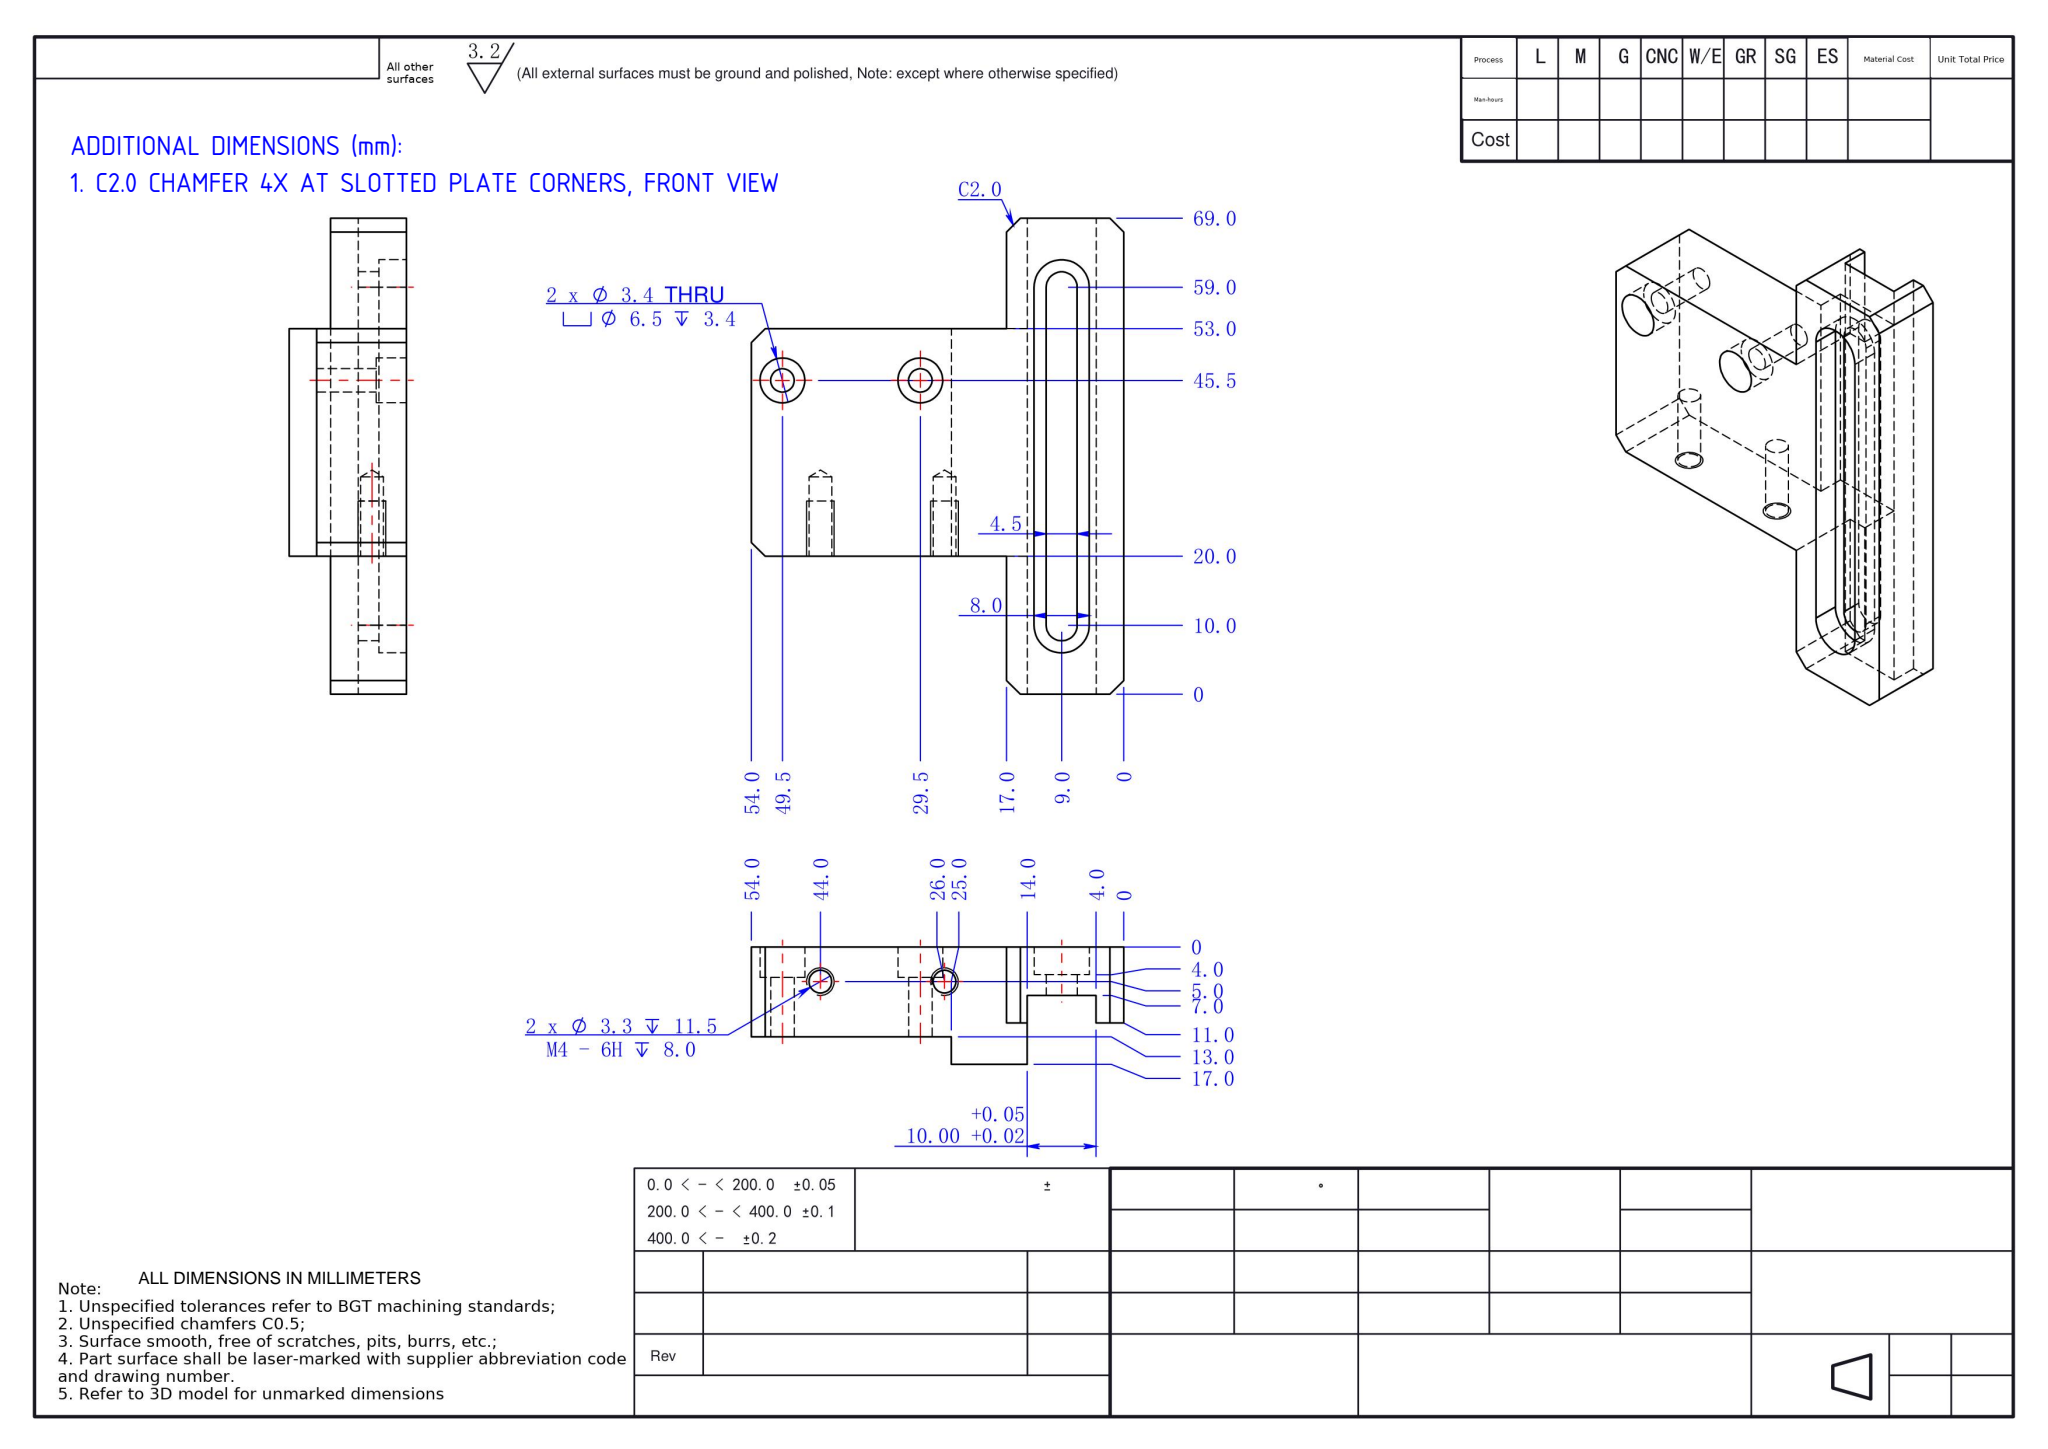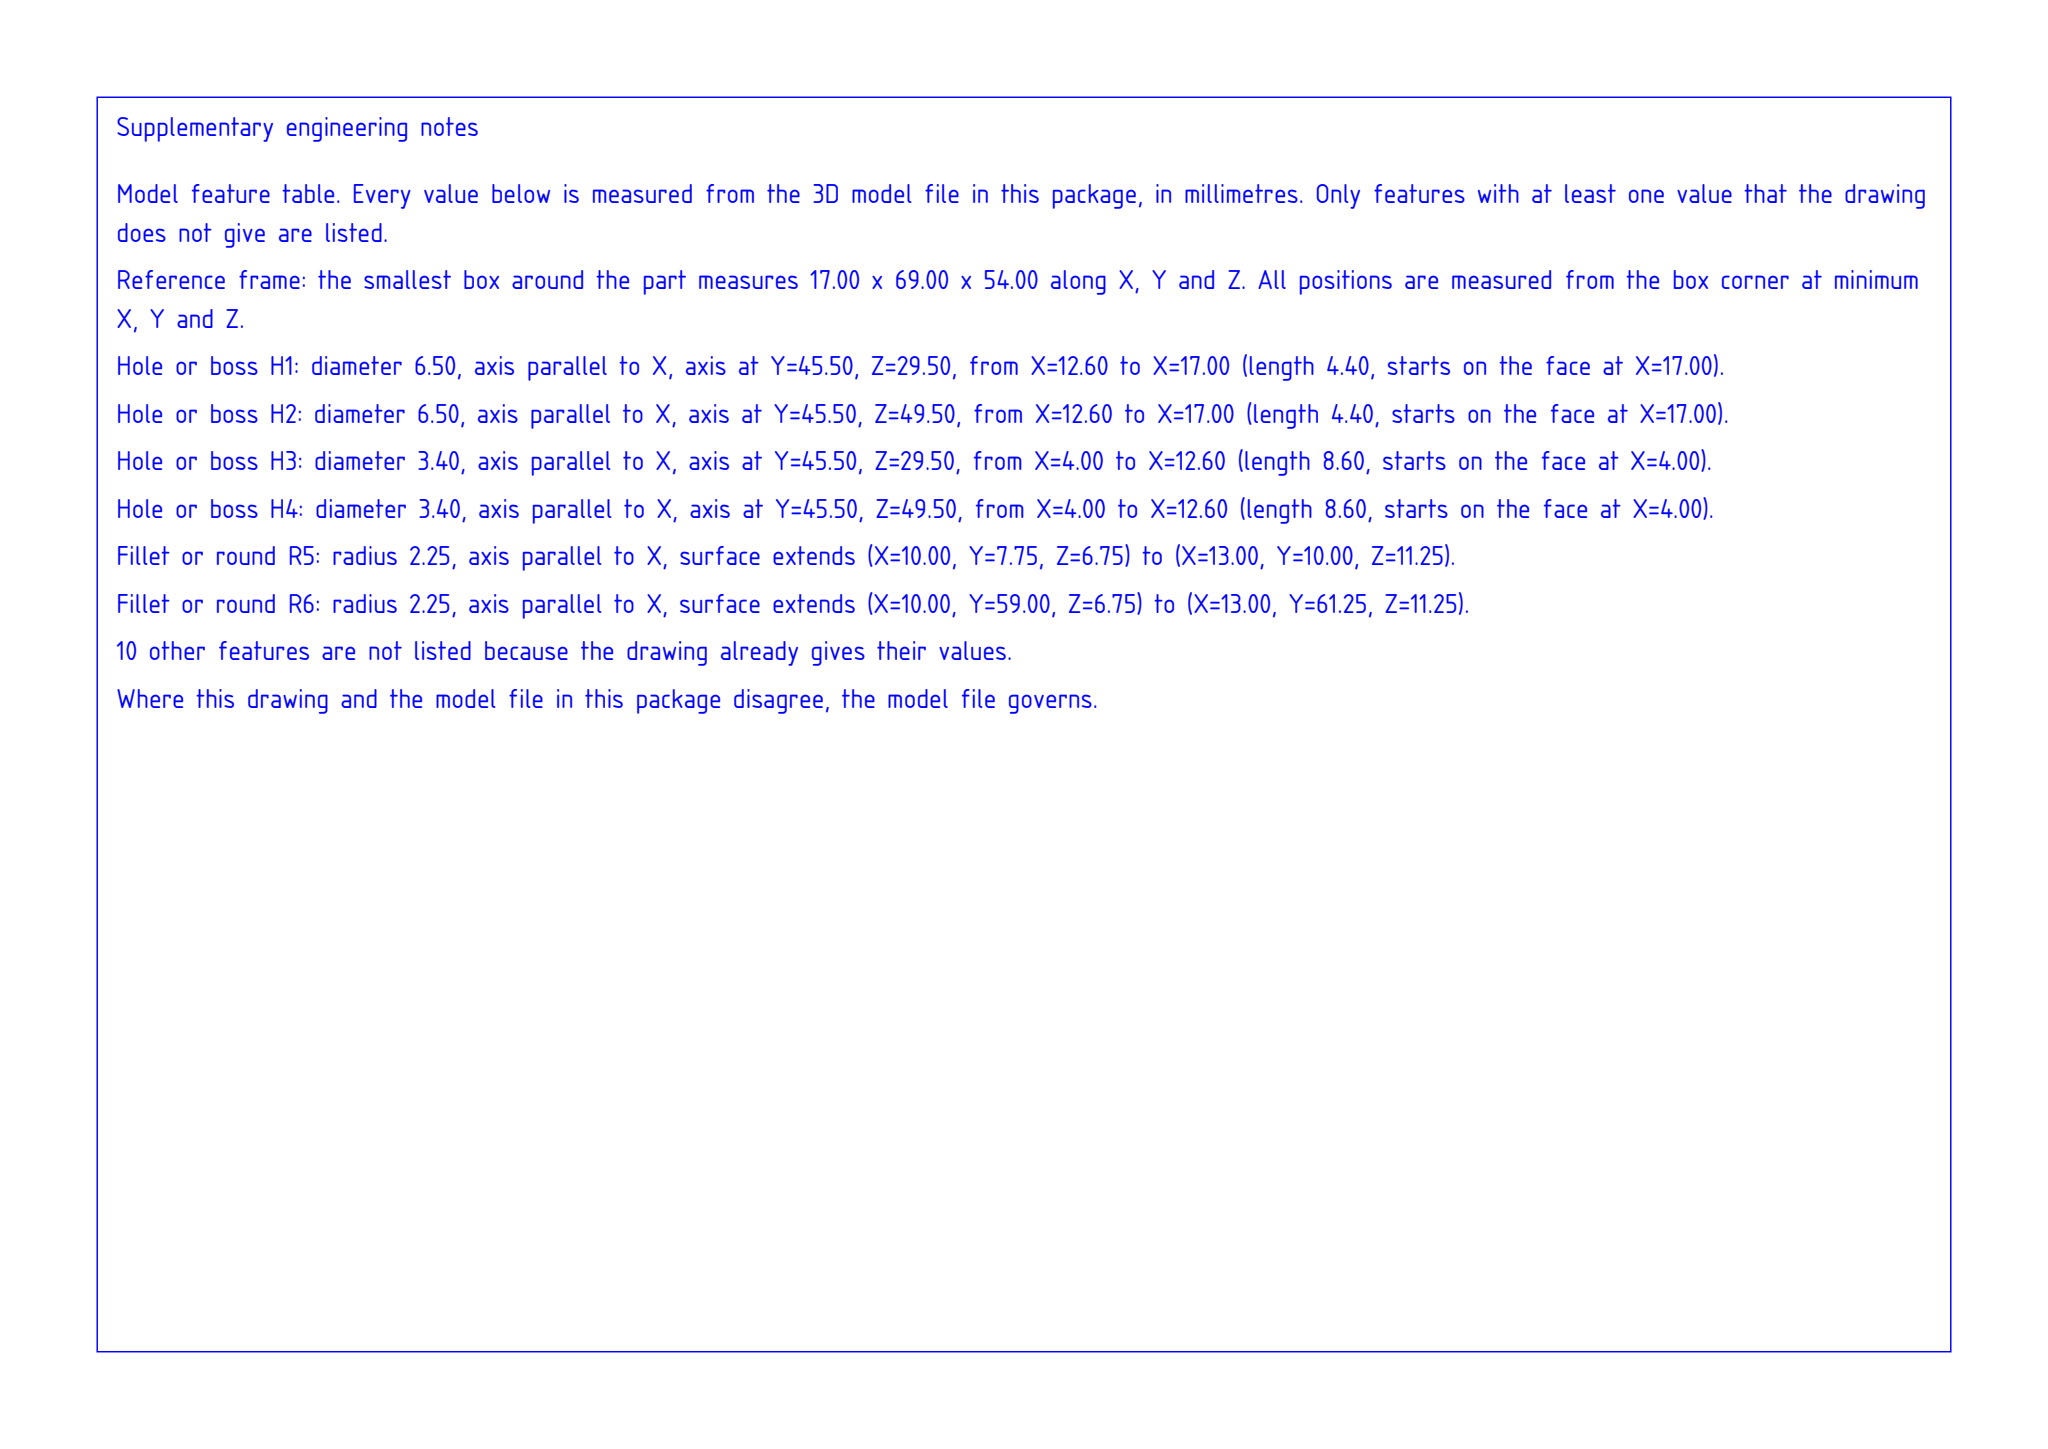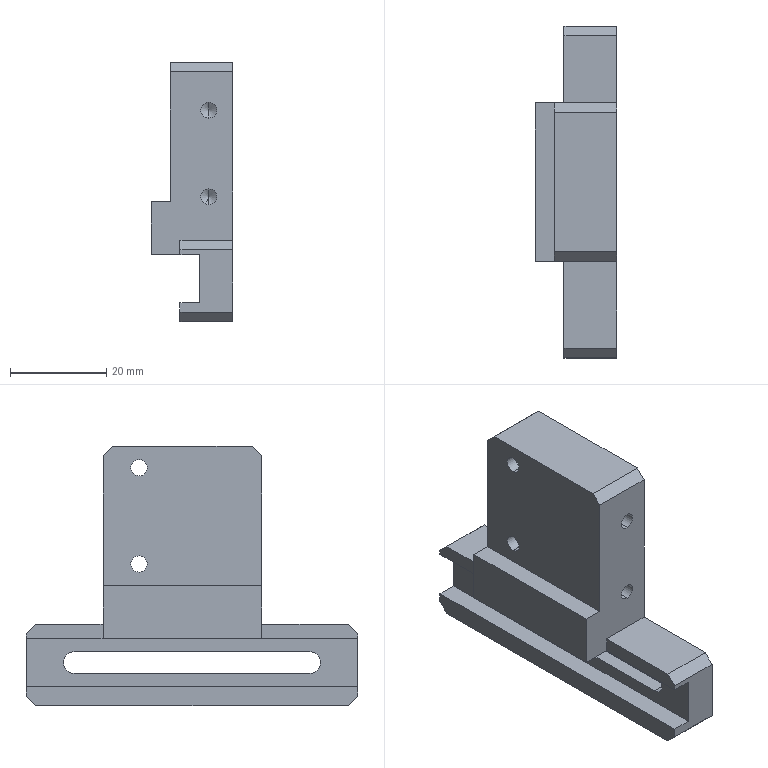Part | SolidWorks | mm | 1 solid | 52 faces | box 17 x 69 x 54 mm | volume 24397 mm3 | plane 31 | cylinder 17 | cone 4 | commonest cylinder face diameters 3.3 x4 6.5 x4 3.4 x4 8 x3 4.5 x2
build123d program:
from build123d import *

# Parameters (mm, degrees)
SKETCH1_W                                       = 16
SKETCH1_H                                       = 50
BOSS_EXTRUDE1_DEPTH                             = 54
SKETCH2_W                                       = 4
SKETCH2_H                                       = 10
CUT_EXTRUDE1_DEPTH                              = 76.151
MOVE_FACE1_BY                                   = 6
SKETCH4_W                                       = 4
SKETCH4_H                                       = 29
CUT_EXTRUDE2_DEPTH                              = 77.592
SKETCH5_W                                       = 22
SKETCH5_H                                       = 21
CUT_EXTRUDE3_DEPTH                              = 192.855
BOSS_EXTRUDE2_DEPTH                             = 20
BOSS_EXTRUDE3_DEPTH                             = 20
SKETCH8_W                                       = 6
SKETCH8_H                                       = 13
CUT_EXTRUDE4_DEPTH                              = 20
SKETCH9_W                                       = 6
SKETCH9_H                                       = 17
CUT_EXTRUDE5_DEPTH                              = 20
MOVE_FACE2_BY                                   = 4
M3_HEX_SOCKET_HEAD_CAP_SCREW_CBORE1_D           = 3.4
M3_HEX_SOCKET_HEAD_CAP_SCREW_CBORE1_CBORE_D     = 6.5
M3_HEX_SOCKET_HEAD_CAP_SCREW_CBORE1_CBORE_DEPTH = 3.4
MOVE_FACE3_BY                                   = 6
MOVE_FACE3_2_BY                                 = 6
SKETCH12_W                                      = 5
SKETCH12_H                                      = 69
CUT_EXTRUDE6_DEPTH                              = 191.903
CHAMFER1_SIZE                                   = 2
CUT_EXTRUDE7_DEPTH                              = 190.983
CUT_EXTRUDE8_DEPTH                              = 4
M4_TAPPED_HOLE1_D                               = 3.3
M4_TAPPED_HOLE1_DEPTH                           = 11.5
M4_TAPPED_HOLE1_TIP                             = 0.9914


with BuildPart() as part:
    # Sketch1 → Boss-Extrude1 (new body)
    with BuildSketch(Plane.XY):
        with Locations((-7.222, -157.872)):
            Rectangle(SKETCH1_W, SKETCH1_H)
    extrude(amount=BOSS_EXTRUDE1_DEPTH)

    # Sketch2 → Cut-Extrude1 (cut, through all)
    with BuildSketch(Plane(origin=(0, -132.872, 0), x_dir=(1, 0, 0), z_dir=(0, 1, 0))):
        with Locations((-13.222, -9)):
            Rectangle(SKETCH2_W, SKETCH2_H)
    extrude(amount=-CUT_EXTRUDE1_DEPTH, mode=Mode.SUBTRACT)

    # Move Face1: a face moved outward by 6.0
    extrude(part.faces().sort_by_distance((-15.222, -157.872, 34))[0], amount=MOVE_FACE1_BY, dir=(-1, 0, 0))

    # Sketch4 → Cut-Extrude2 (cut, through all)
    with BuildSketch(Plane(origin=(0, -132.872, 0), x_dir=(1, 0, 0), z_dir=(0, 1, 0))):
        with Locations((-19.222, -39.5)):
            Rectangle(SKETCH4_W, SKETCH4_H)
    extrude(amount=-CUT_EXTRUDE2_DEPTH, mode=Mode.SUBTRACT)

    # Sketch5 → Cut-Extrude3 (cut, through all)
    with BuildSketch(Plane.XY.offset(54)):
        with Locations((-10.222, -172.372)):
            Rectangle(SKETCH5_W, SKETCH5_H)
    extrude(amount=-CUT_EXTRUDE3_DEPTH, mode=Mode.SUBTRACT)

    # Sketch6 → Boss-Extrude2 (add)
    with BuildSketch(Plane(origin=(0, -132.872, 0), x_dir=(1, 0, 0), z_dir=(0, 1, 0))):
        Polygon((-11.222, -4), (-15.222, -4), (-15.222, 0), (0.7776, 0), (0.7776, -17), (-21.222, -17), (-21.222, -14), (-11.222, -14), align=None)
    extrude(amount=BOSS_EXTRUDE2_DEPTH)

    # Sketch7 → Boss-Extrude3 (add)
    with BuildSketch(Plane.XZ.offset(161.872)):
        Polygon((0.7776, 17), (0.7776, 0), (-15.222, 0), (-15.222, 4), (-11.222, 4), (-11.222, 14), (-21.222, 14), (-21.222, 17), align=None)
    extrude(amount=BOSS_EXTRUDE3_DEPTH)

    # Sketch8 → Cut-Extrude4 (cut)
    with BuildSketch(Plane(origin=(0, -112.872, 0), x_dir=(1, 0, 0), z_dir=(0, 1, 0))):
        with Locations((-18.222, -10.5)):
            Rectangle(SKETCH8_W, SKETCH8_H)
    extrude(amount=-CUT_EXTRUDE4_DEPTH, mode=Mode.SUBTRACT)

    # Sketch9 → Cut-Extrude5 (cut)
    with BuildSketch(Plane.XZ.offset(181.872)):
        with Locations((-18.222, 8.5)):
            Rectangle(SKETCH9_W, SKETCH9_H)
    extrude(amount=-CUT_EXTRUDE5_DEPTH, mode=Mode.SUBTRACT)

    # Move Face2: a face moved outward by 4.0
    extrude(part.faces().sort_by_distance((-8.965, -132.872, 34.349))[0], amount=MOVE_FACE2_BY, dir=(0, 1, 0))

    # M3 Hex Socket Head Cap Screw CBORE1 (through all)
    with Locations(Plane(origin=(0.7776, 0, 0), x_dir=(0, 0, -1), z_dir=(1, 0, 0))):
        with Locations((-49.5, -136.372), (-29.5, -136.372)):
            CounterBoreHole(M3_HEX_SOCKET_HEAD_CAP_SCREW_CBORE1_D / 2, M3_HEX_SOCKET_HEAD_CAP_SCREW_CBORE1_CBORE_D / 2, M3_HEX_SOCKET_HEAD_CAP_SCREW_CBORE1_CBORE_DEPTH)

    # Move Face3: a face moved inward by 6.0
    extrude(part.faces().sort_by_distance((-2.622, -138.972, 49.5))[0], amount=MOVE_FACE3_BY, dir=(-1, 0, 0), mode=Mode.SUBTRACT)

    # Move Face3 2: a face moved inward by 6.0
    extrude(part.faces().sort_by_distance((-2.622, -138.972, 29.5))[0], amount=MOVE_FACE3_2_BY, dir=(-1, 0, 0), mode=Mode.SUBTRACT)

    # Sketch12 → Cut-Extrude6 (cut, through all)
    with BuildSketch(Plane.XY.offset(54)):
        with Locations((-1.722, -147.372)):
            Rectangle(SKETCH12_W, SKETCH12_H)
    extrude(amount=-CUT_EXTRUDE6_DEPTH, mode=Mode.SUBTRACT)

    # Chamfer1
    chamfer1_edges = [part.edges().sort_by_distance(p)[0] for p in [
        (-9.722, -181.872, 0),
        (-9.722, -112.872, 17),
        (-9.722, -181.872, 17),
        (-9.722, -112.872, 0),
        (-10.722, -161.872, 54),
        (-10.722, -128.872, 54),
    ]]
    chamfer(chamfer1_edges, length=CHAMFER1_SIZE)

    # Sketch13 → Cut-Extrude7 (cut, through all)
    with BuildSketch(Plane.ZY.offset(11.222)):
        with BuildLine():
            Line((11.25, -122.872), (11.25, -171.872))
            ThreePointArc((11.25, -171.872), (9, -174.122), (6.75, -171.872))
            Line((6.75, -171.872), (6.75, -122.872))
            ThreePointArc((6.75, -122.872), (9, -120.622), (11.25, -122.872))
        make_face()
    extrude(amount=-CUT_EXTRUDE7_DEPTH, mode=Mode.SUBTRACT)

    # Sketch14 → Cut-Extrude8 (cut)
    with BuildSketch(Plane(origin=(-4.222, 0, 0), x_dir=(0, 0, -1), z_dir=(1, 0, 0))):
        with BuildLine():
            Line((-5, -122.872), (-5, -171.872))
            ThreePointArc((-5, -171.872), (-9, -175.872), (-13, -171.872))
            Line((-13, -171.872), (-13, -122.872))
            ThreePointArc((-13, -122.872), (-9, -118.872), (-5, -122.872))
        make_face()
    extrude(amount=-CUT_EXTRUDE8_DEPTH, mode=Mode.SUBTRACT)

    # M4 Tapped Hole1
    with Locations(Plane(origin=(0, -161.872, 0), x_dir=(-1, 0, 0), z_dir=(0, -1, 0))):
        with Locations((9.222, -44), (9.222, -26)):
            Hole(M4_TAPPED_HOLE1_D / 2, depth=M4_TAPPED_HOLE1_DEPTH)
            with Locations((0, 0, -(M4_TAPPED_HOLE1_DEPTH + M4_TAPPED_HOLE1_TIP / 2))):  # 118° drill point
                Cone(0, M4_TAPPED_HOLE1_D / 2, M4_TAPPED_HOLE1_TIP, mode=Mode.SUBTRACT)


solid = part.part